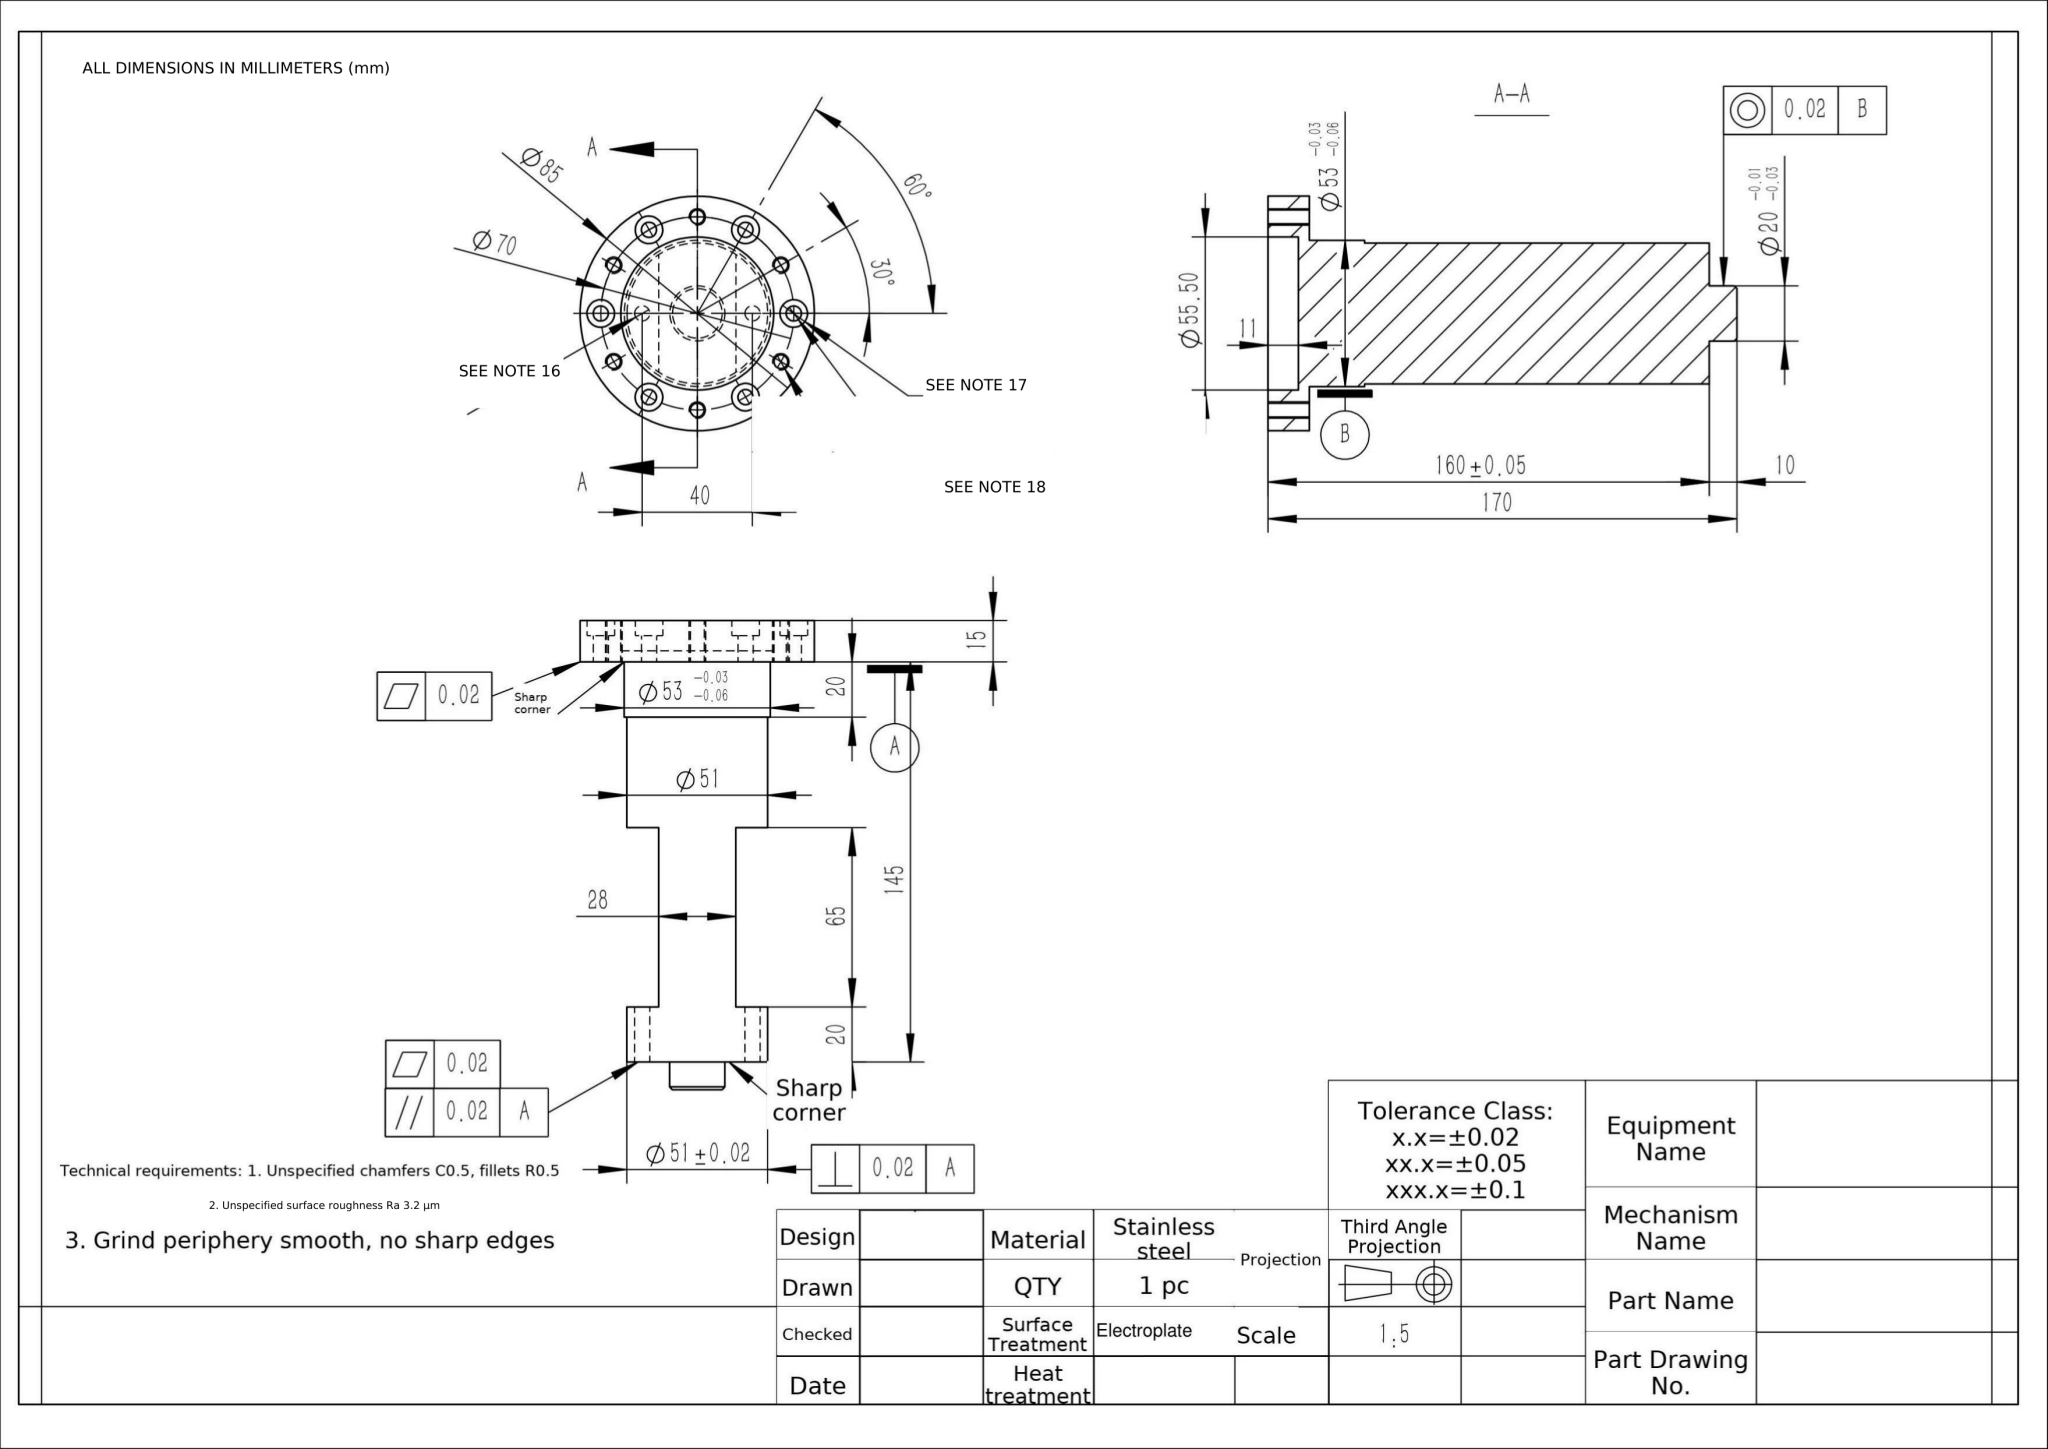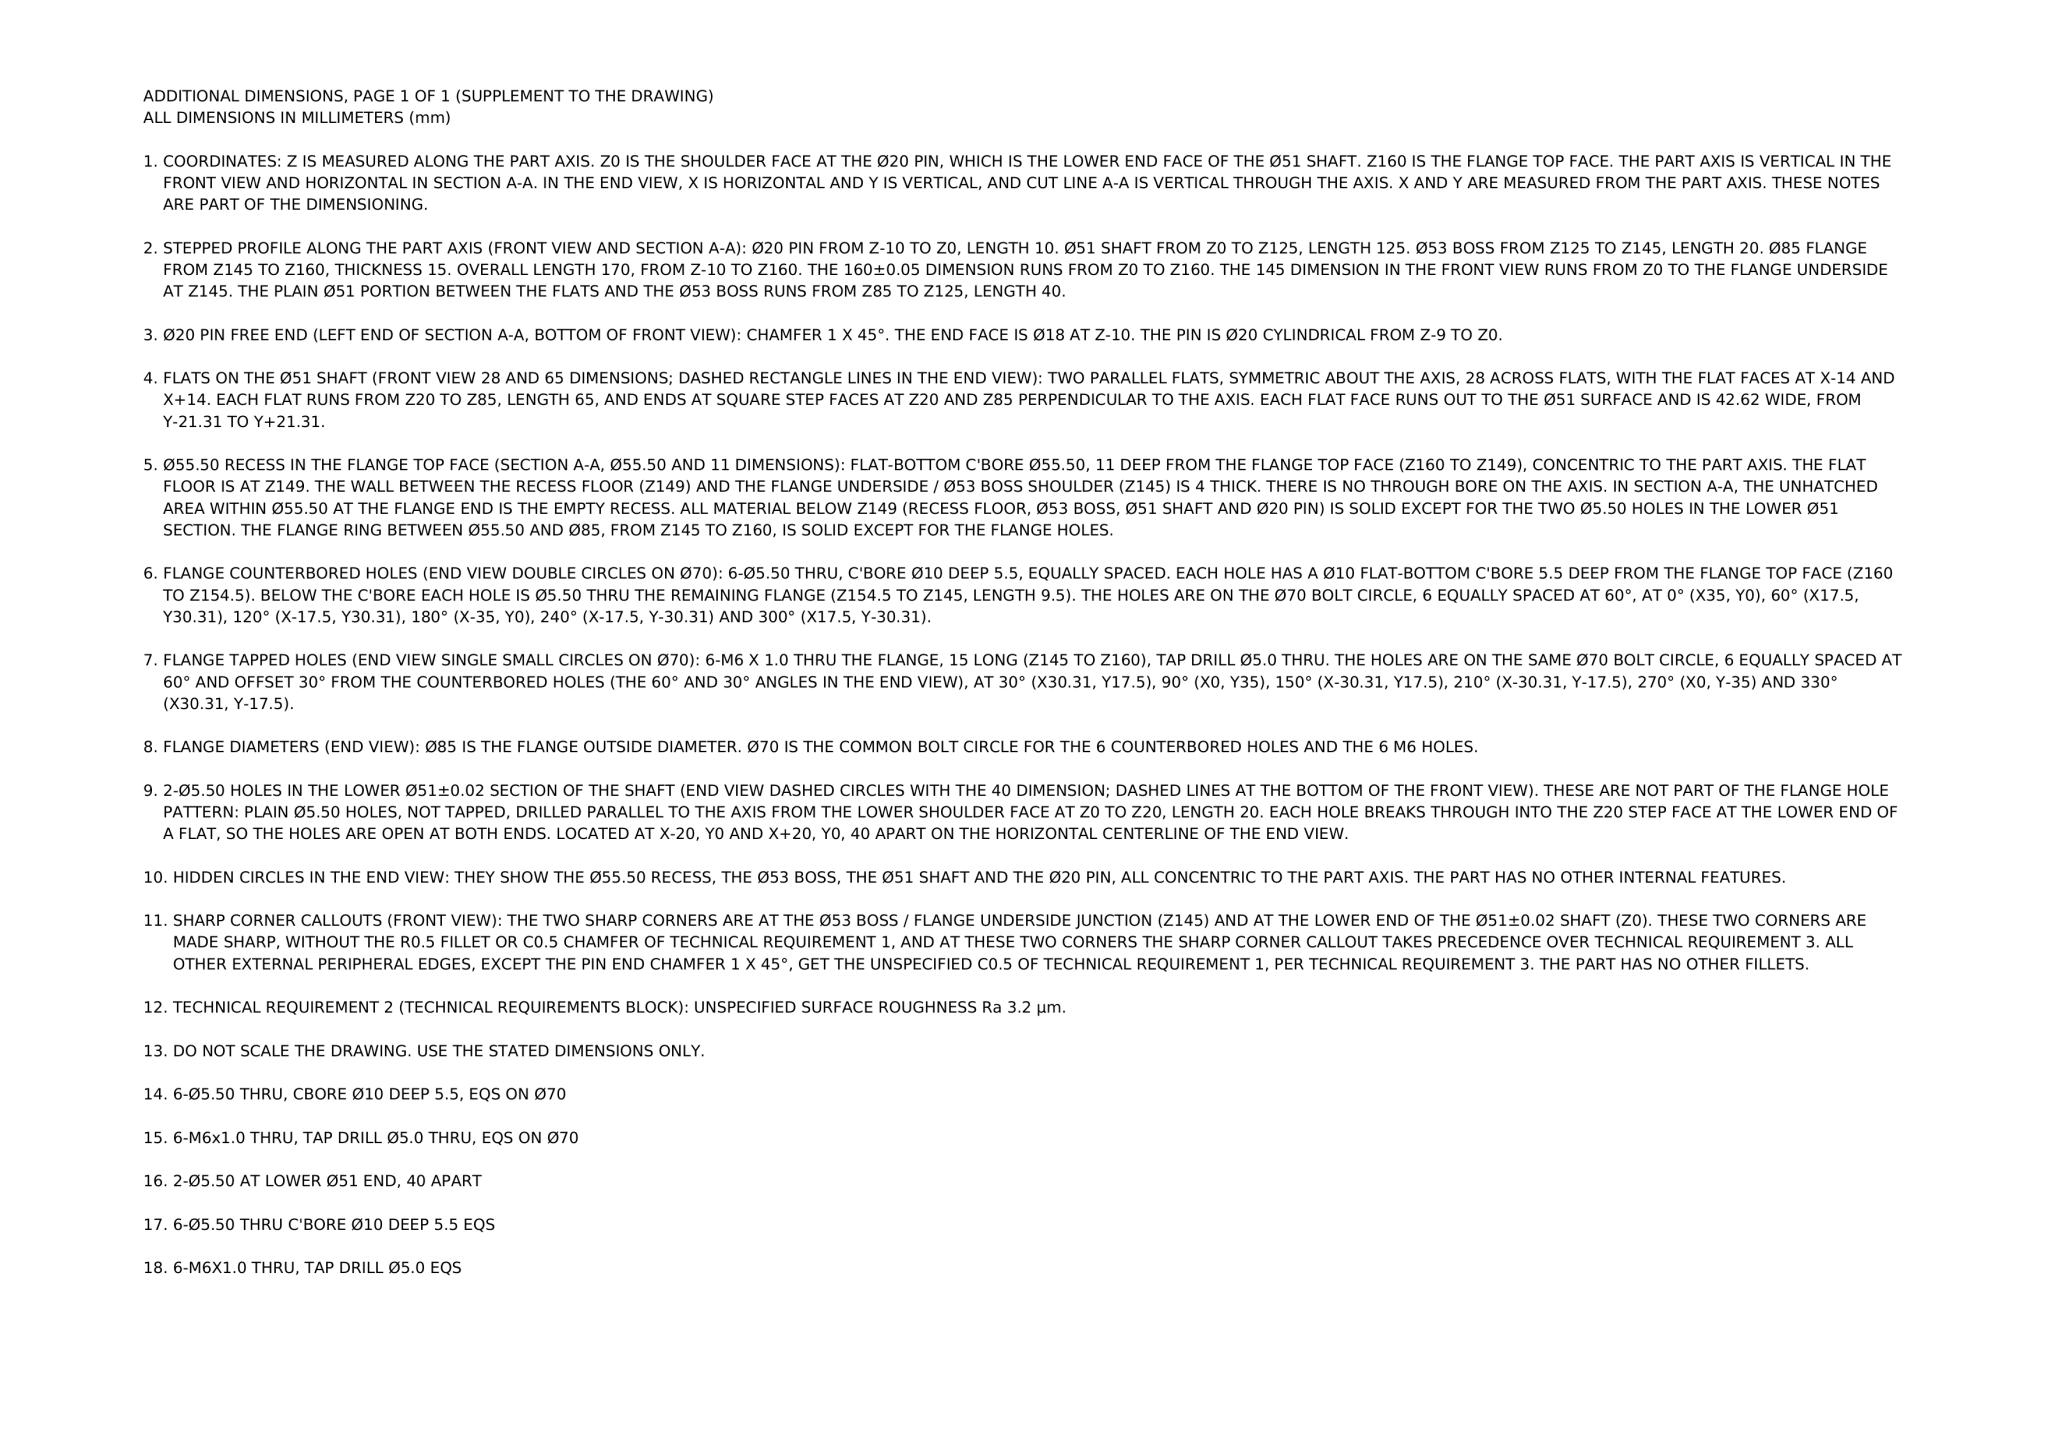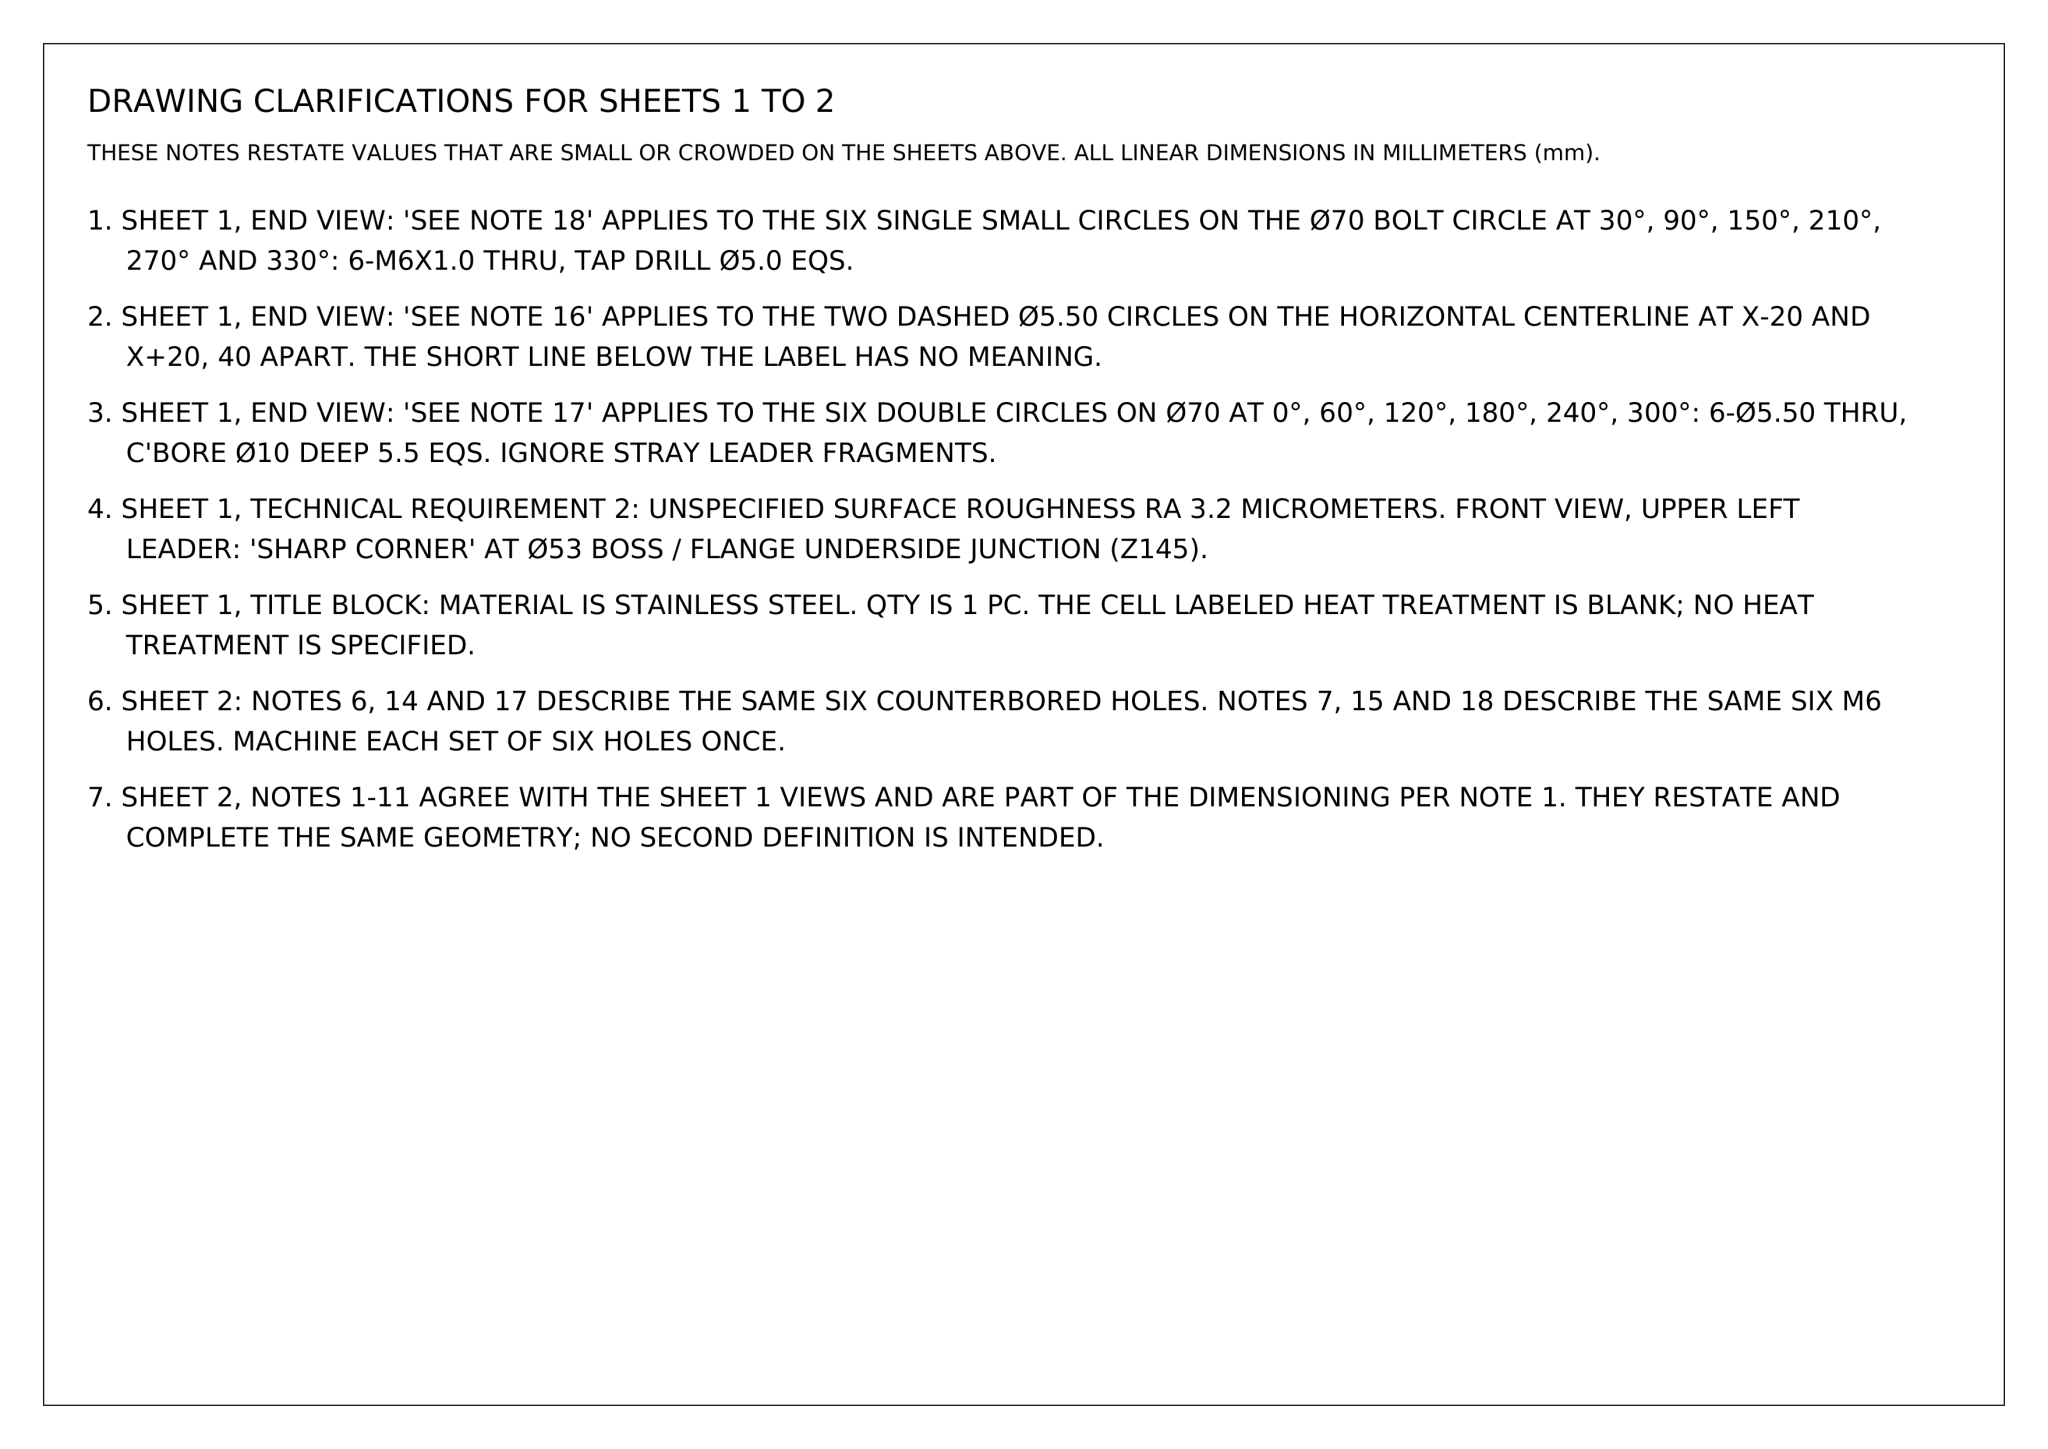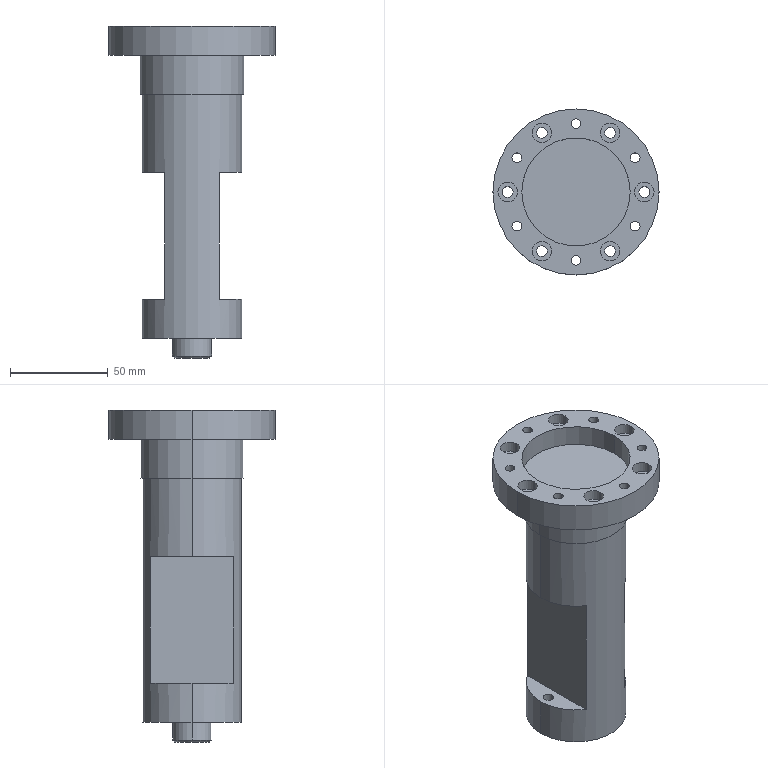Part | NX | mm | 1 solid | 70 faces | box 85 x 85 x 170 mm | volume 309566 mm3 | cylinder 50 | plane 18 | cone 2 | commonest cylinder face diameters 5.5 x16 5 x12 10 x12 20 x2 51 x2 53 x2 55.5 x2 85 x2